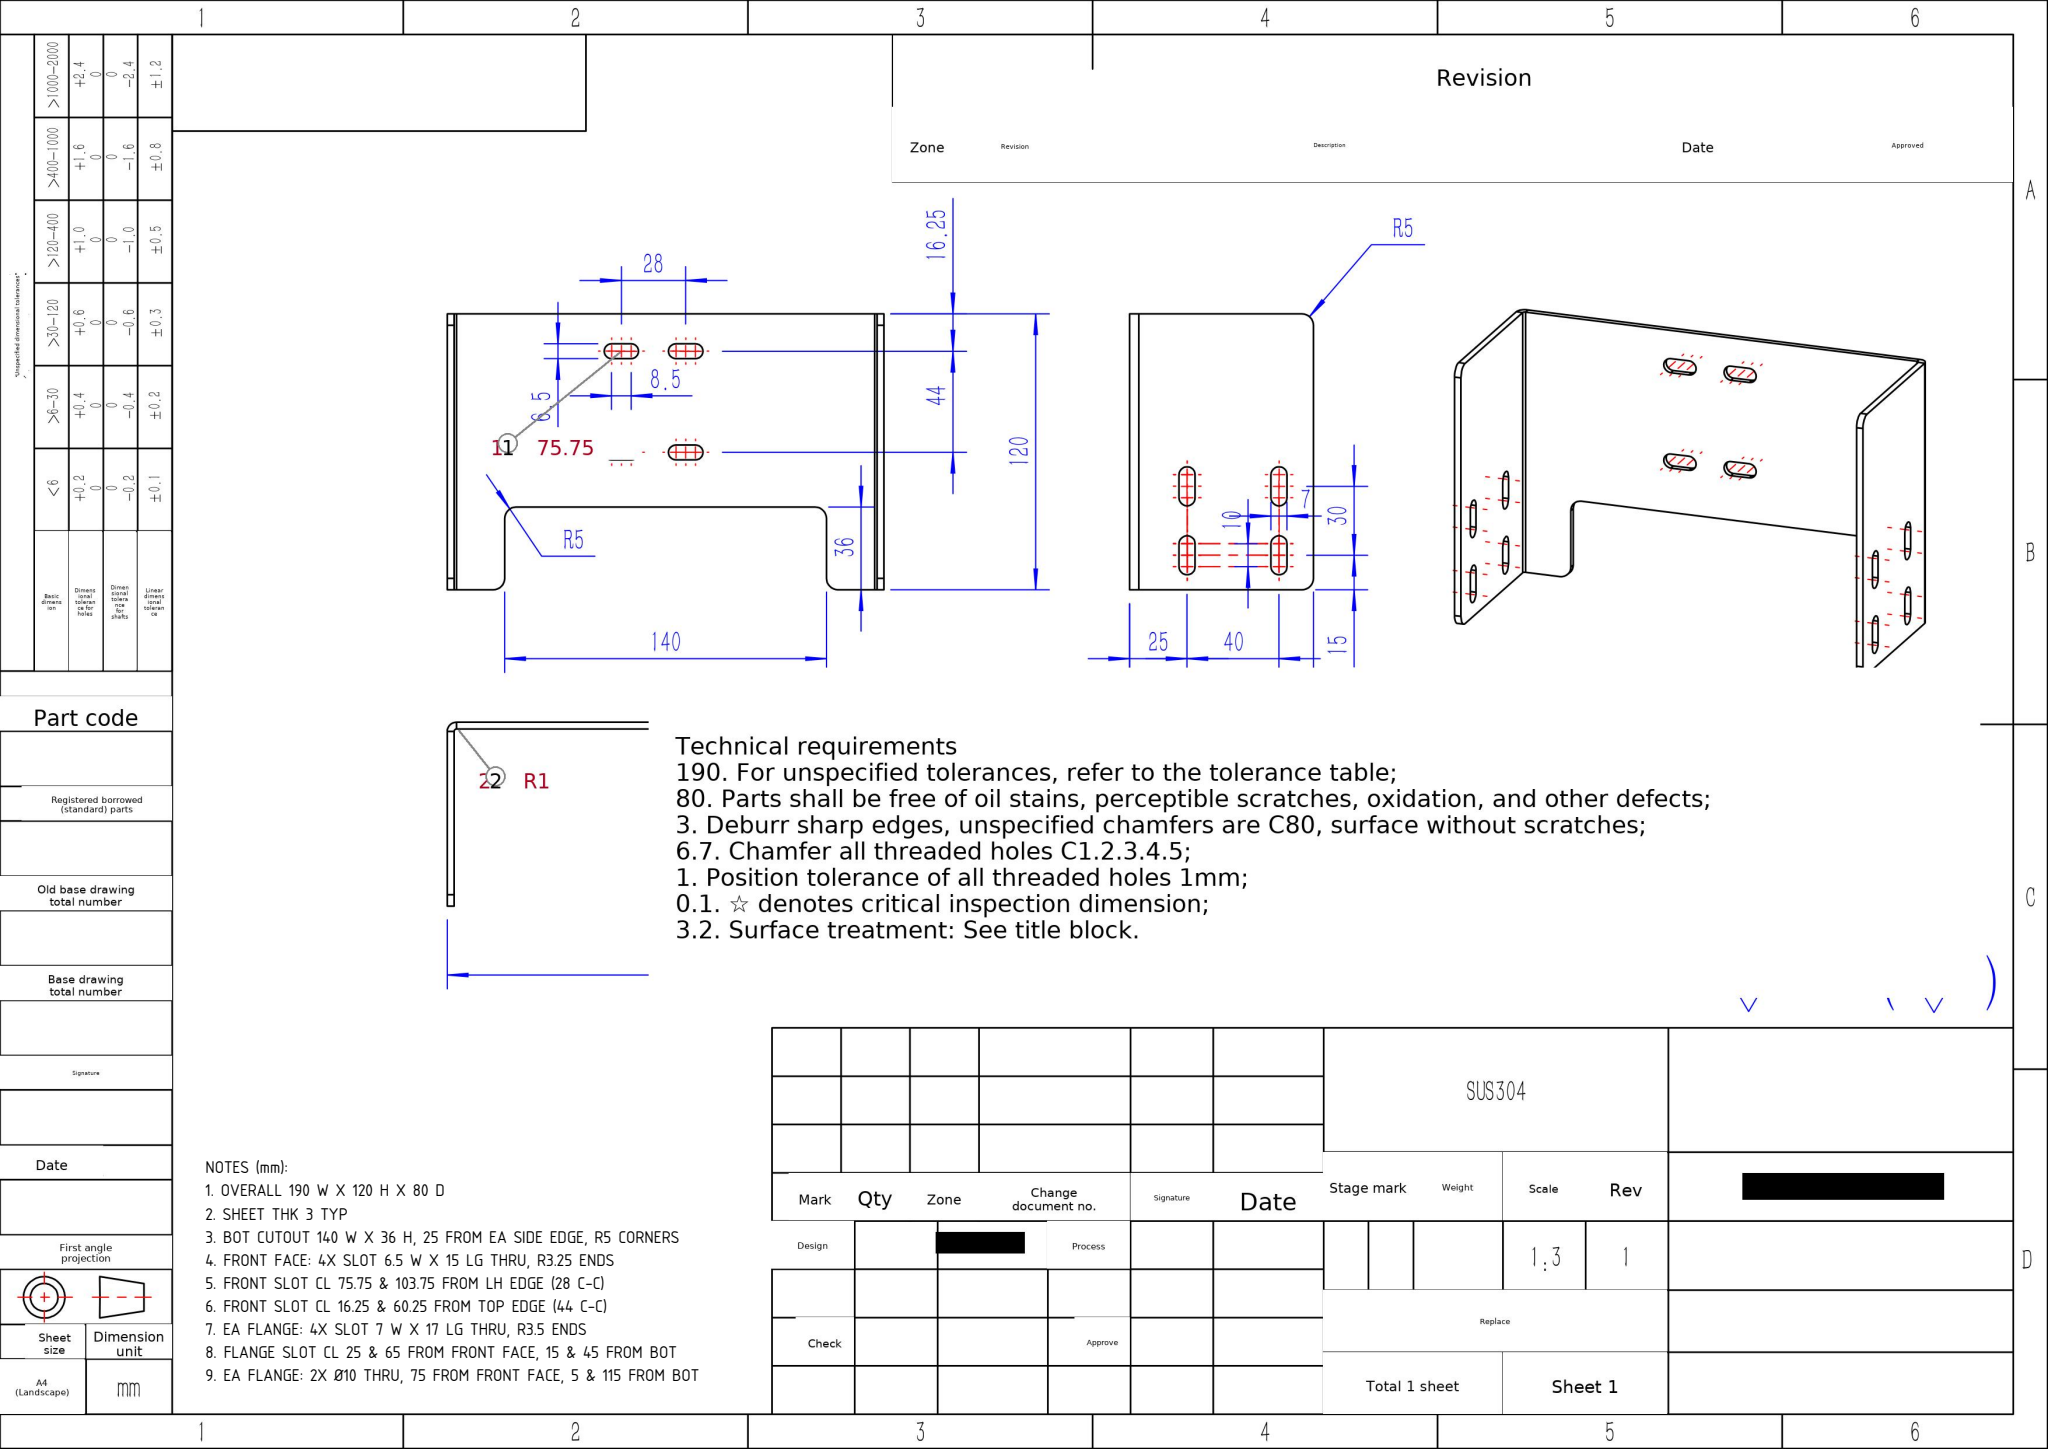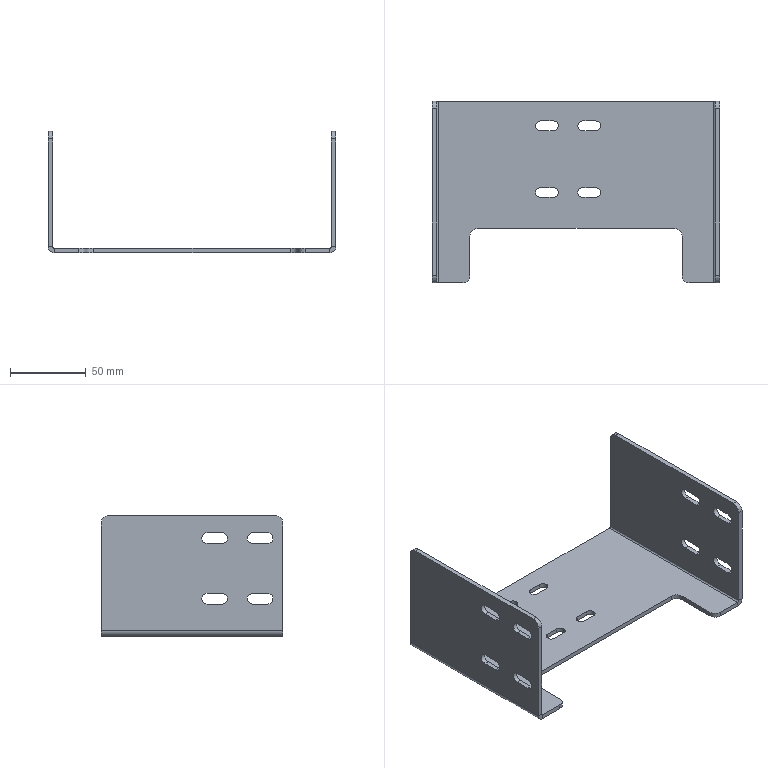Part | SolidWorks | mm | 1 solid | 86 faces | box 190 x 120 x 80 mm | volume 104218 mm3 | plane 46 | cylinder 40 | commonest cylinder face diameters 7 x16 6.5 x12 10 x8 2 x2 8 x2
Drawing notes:
OVERALL 190 W X 120 H X 80 D | from the solid: bbox_xyz 190 x 120 x 80
SHEET THK 3 TYP | from the solid: z planes 0 & 3 (front panel), x planes 0/3 & 187/190 (flanges) => 3 mm wall
BOT CUTOUT 140 W X 36 H, 25 FROM EA SIDE EDGE, R5 CORNERS | from the solid: x planes 25 & 165 (140 wide, 25 from x=0/190), y plane 36; R5 corner cyls at (30,31),(160,31)
FRONT FACE: 4X SLOT 6.5 W X 15 LG THRU, R3.25 ENDS | from the solid: Ø6.5 z-axis cyls paired 71.5/80 and 99.5/108, len 3; 8.5 c-c + 6.5 = 15 lg
FRONT SLOT CL 75.75 & 103.75 FROM LH EDGE (28 C-C) | from the solid: slot end centers x=71.5/80 -> CL 75.75; x=99.5/108 -> CL 103.75; bbox x 0-190
FRONT SLOT CL 16.25 & 60.25 FROM TOP EDGE (44 C-C) | from the solid: slot y=103.75 & 59.75 from min corner; bbox y=120 -> 16.25 & 60.25 from top
EA FLANGE: 4X SLOT 7 W X 17 LG THRU, R3.5 ENDS | from the solid: Ø7 x-axis cyls paired y=10/20 and y=40/50, len 3; 10 c-c + 7 = 17 lg
FLANGE SLOT CL 25 & 65 FROM FRONT FACE, 15 & 45 FROM BOT | from the solid: Ø7 slots at z=25 & 65; CL y=(10+20)/2=15 and (40+50)/2=45; front face z=0
EA FLANGE: 2X Ø10 THRU, 75 FROM FRONT FACE, 5 & 115 FROM BOT | from the solid: Ø10 x-axis cyls at (y=5,z=75) and (y=115,z=75), len 3, count 2 ea